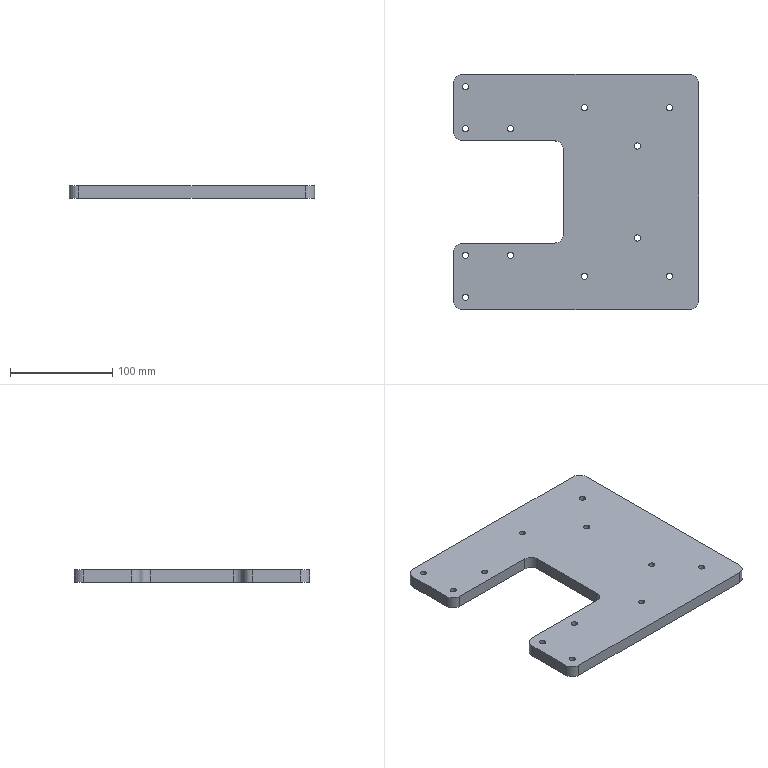Component | NX | BASE_PLATE_1 | 1 solid | 30 faces | volume 527894 mm3 | cylinder 20 | plane 10 | commonest cylinder face diameters 6 x12 18 x8